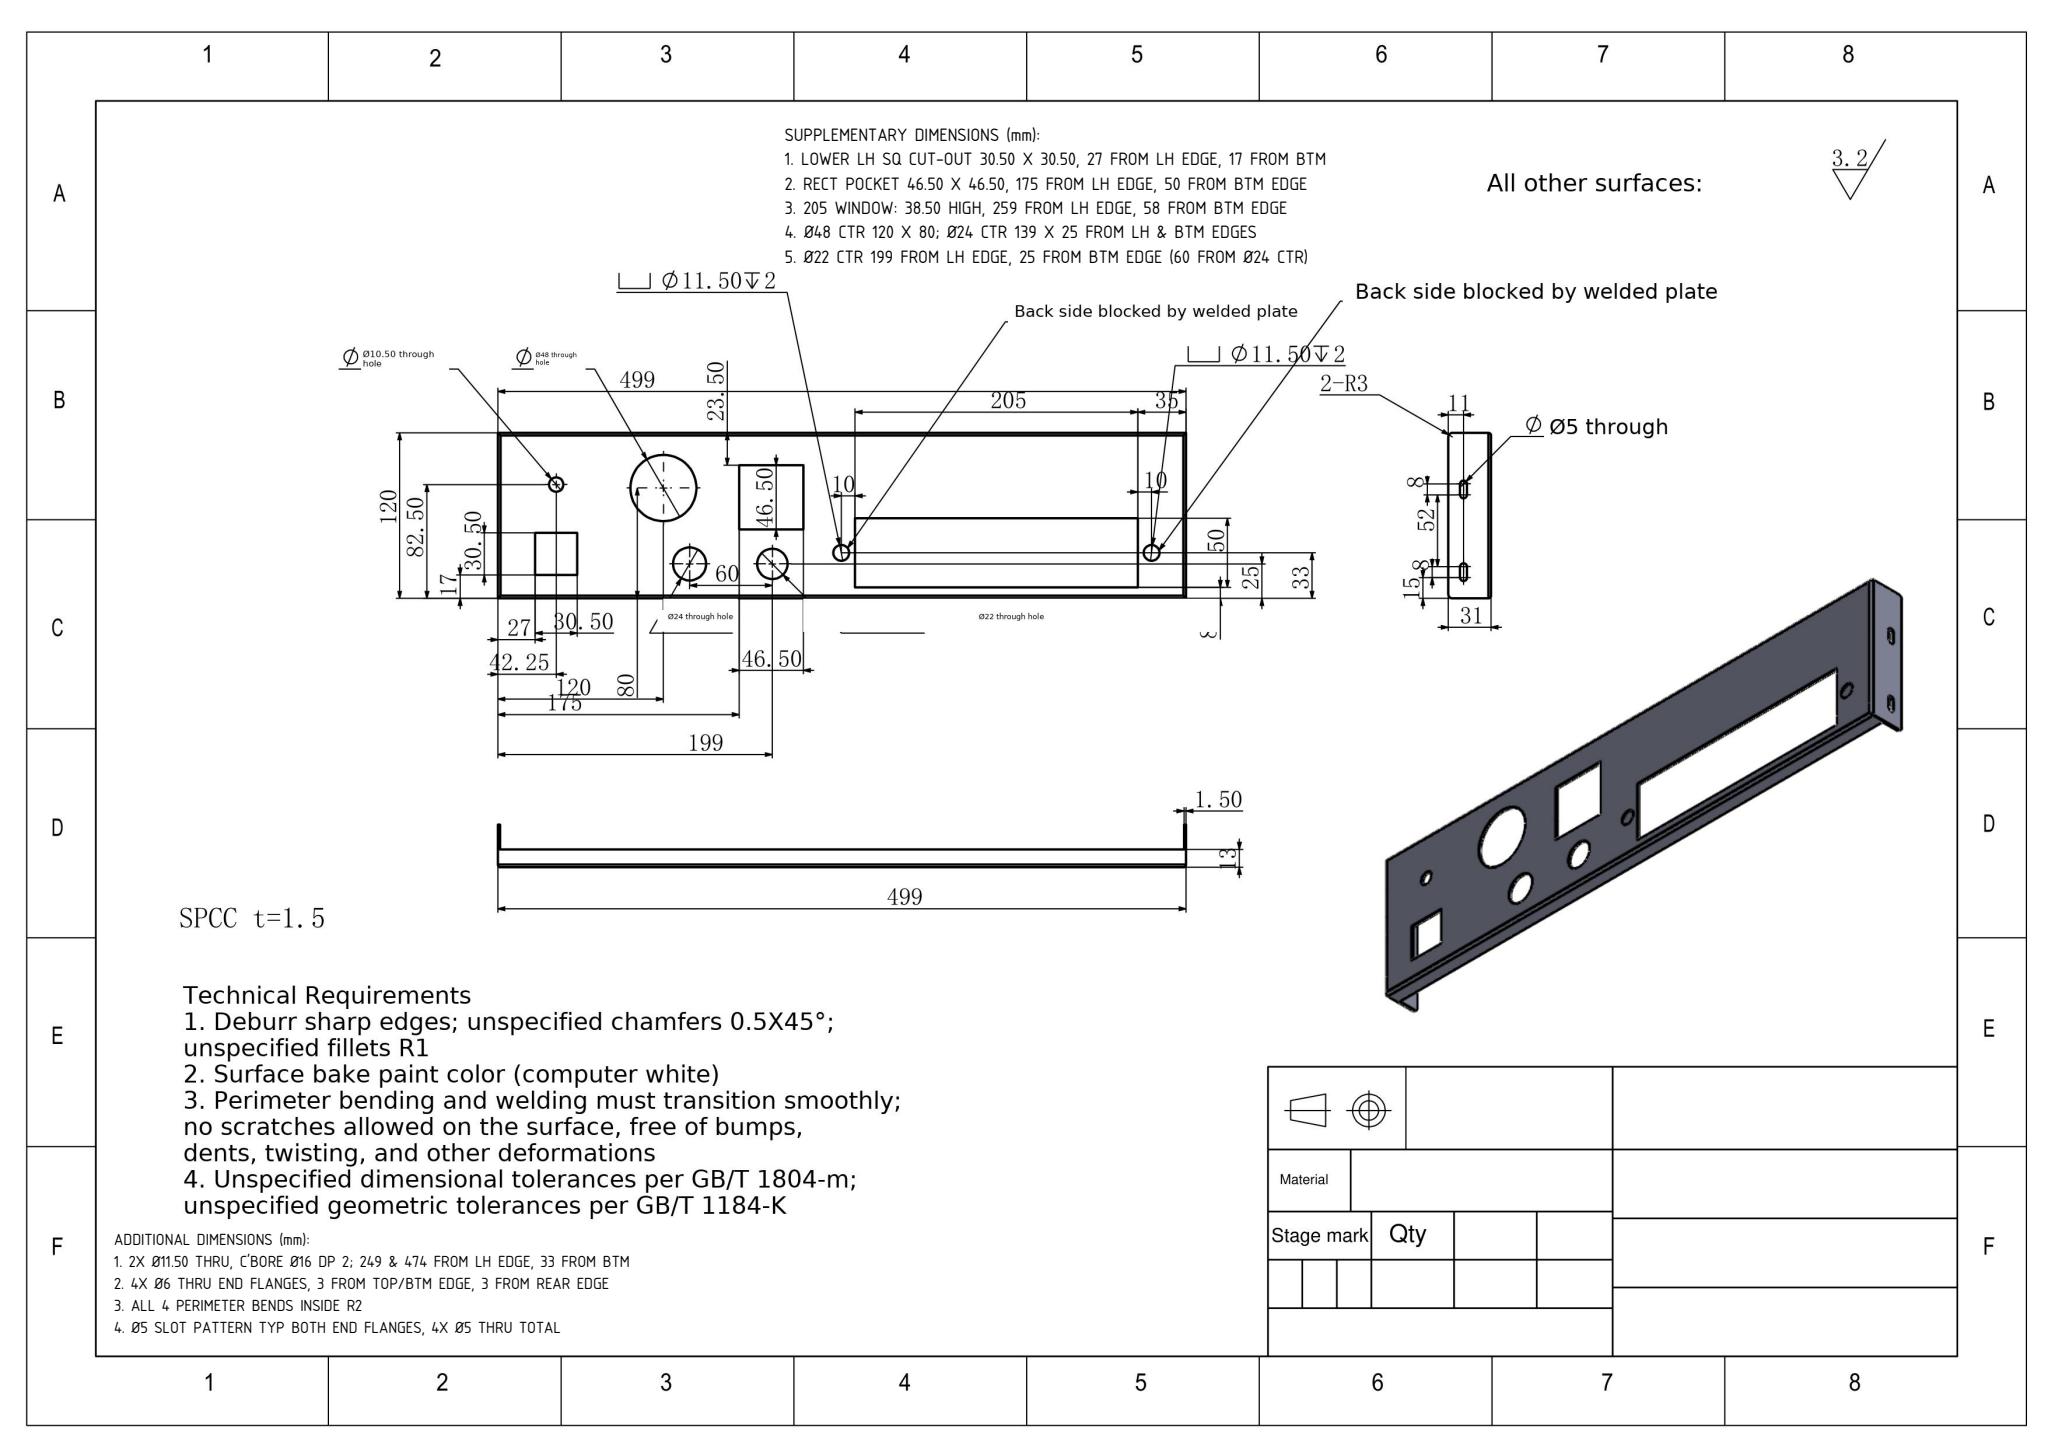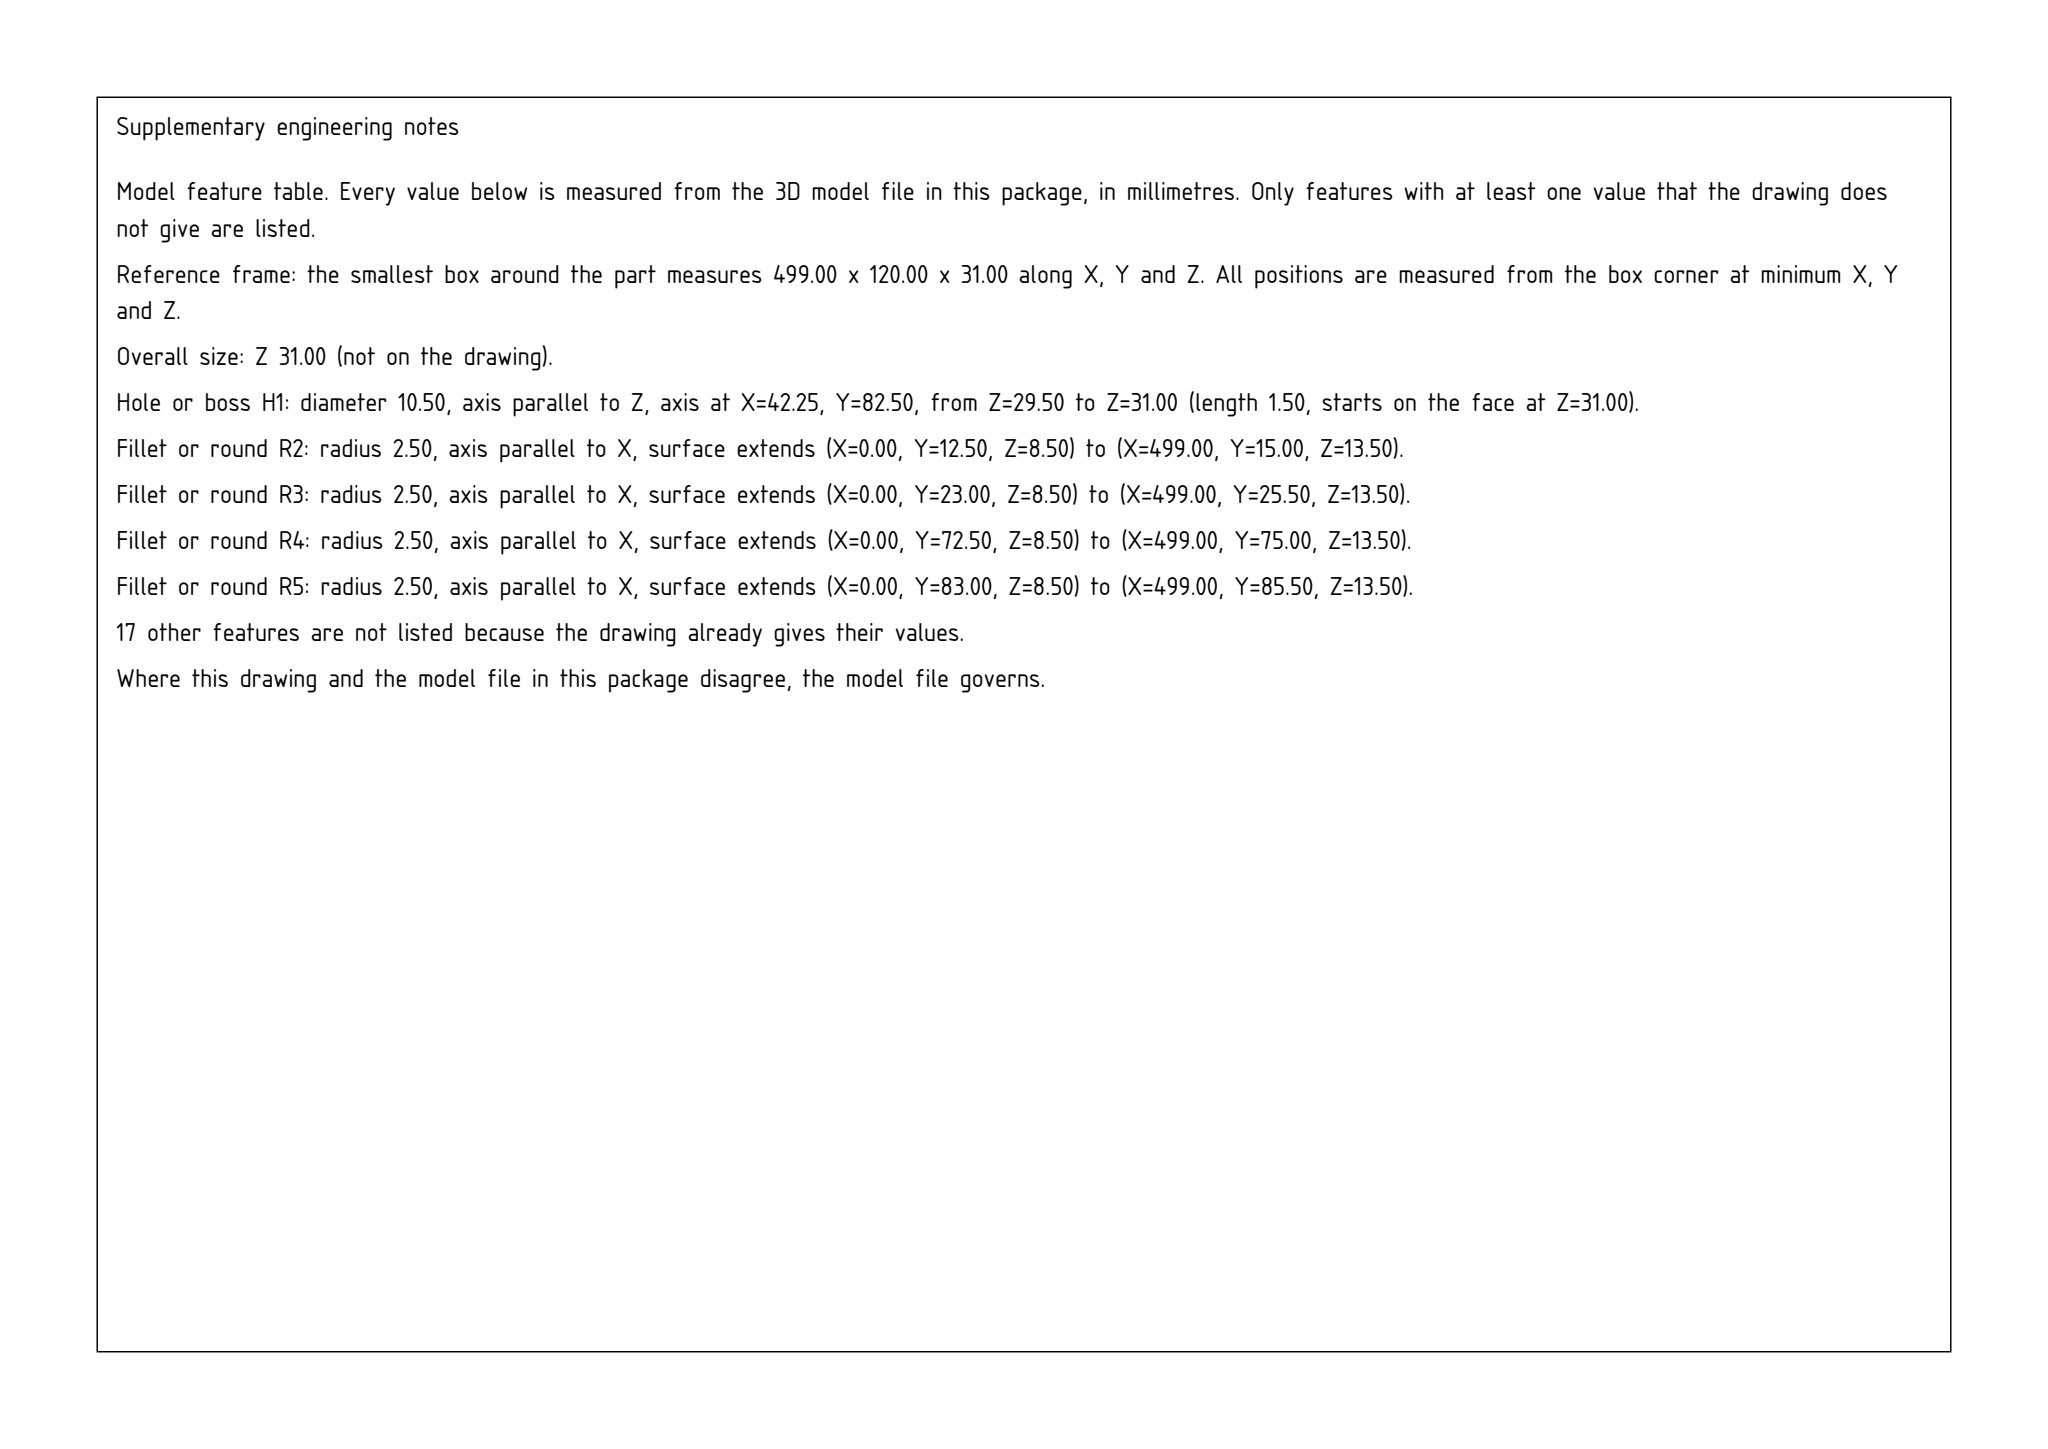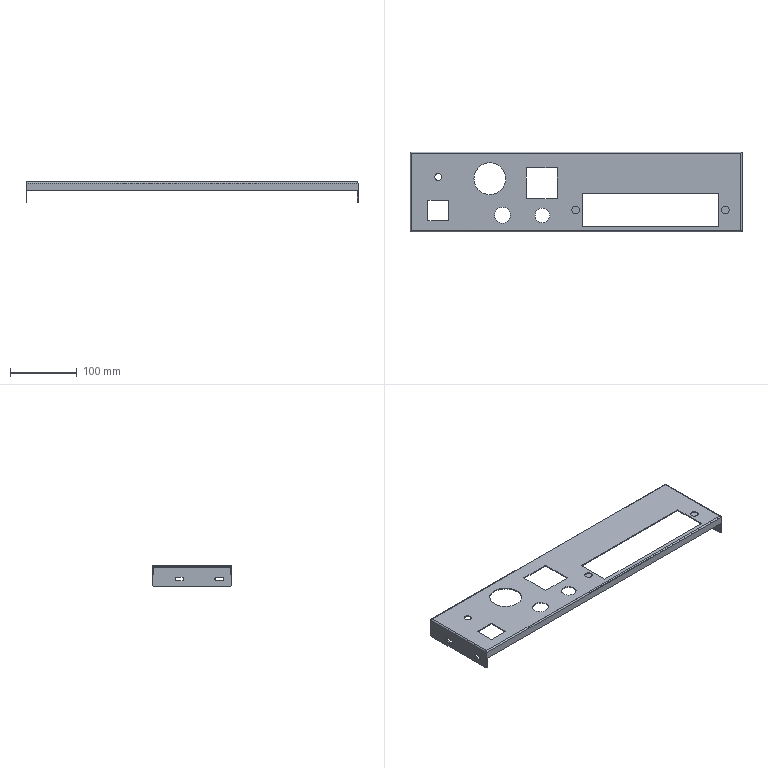Part | SolidWorks | mm | 1 solid | 74 faces | box 499 x 120 x 31 mm | volume 92575 mm3 | plane 38 | cylinder 36 | commonest cylinder face diameters 5 x8 16 x4 11.5 x4 1 x4 4 x4 6 x4 22 x2 24 x2
build123d program:
from build123d import *

# Parameters (mm, degrees)
SKETCH1_W           = 499
SKETCH1_H           = 120
BOSS_EXTRUDE1_DEPTH = 31
SKETCH2_W           = 496
SKETCH2_H           = 15
CUT_EXTRUDE1_DEPTH  = 451.195
SKETCH3_W           = 496
SKETCH3_H           = 96
CUT_EXTRUDE2_DEPTH  = 14.5
SKETCH4_W           = 496
SKETCH4_H           = 13
CUT_EXTRUDE3_DEPTH  = 10.5
SKETCH5_W           = 496
SKETCH5_H           = 13
CUT_EXTRUDE4_DEPTH  = 10.5
CUT_EXTRUDE5_DEPTH  = 620.957
CUT_EXTRUDE6_REACH  = 623.162
CUT_EXTRUDE7_DEPTH  = 620.957
CUT_EXTRUDE8_DEPTH  = 622.162
FILLET1_R           = 0.5
FILLET2_R           = 2
FILLET3_R           = 3
SKETCH10_R          = 5.25
SKETCH10_R_2        = 24
SKETCH10_R_3        = 12
SKETCH10_R_4        = 11
SKETCH10_W          = 30.5
SKETCH10_H          = 30.5
SKETCH10_W_2        = 46.5
SKETCH10_H_2        = 46.5
CUT_EXTRUDE9_DEPTH  = 273.079
SKETCH11_W          = 496
SKETCH11_H          = 120
CUT_EXTRUDE10_DEPTH = 3
SKETCH12_W          = 205
SKETCH12_H          = 50
CUT_EXTRUDE11_DEPTH = 273.079
SKETCH13_R          = 5.75
CUT_EXTRUDE12_DEPTH = 273.079
SKETCH14_R          = 8
BOSS_EXTRUDE2_DEPTH = 2


with BuildPart() as part:
    # Sketch1 → Boss-Extrude1 (new body)
    with BuildSketch(Plane(origin=(0, 0, 324), x_dir=(-1, 0, 0), z_dir=(0, 0, -1))):
        with Locations((0, -44)):
            Rectangle(SKETCH1_W, SKETCH1_H)
    extrude(amount=-BOSS_EXTRUDE1_DEPTH)

    # Sketch2 → Cut-Extrude1 (cut, through all)
    with BuildSketch(Plane(origin=(0, 16, 0), x_dir=(-1, 0, 0), z_dir=(0, 1, 0))):
        with Locations((0, 331.5)):
            Rectangle(SKETCH2_W, SKETCH2_H)
    extrude(amount=-CUT_EXTRUDE1_DEPTH, mode=Mode.SUBTRACT)

    # Sketch3 → Cut-Extrude2 (cut)
    with BuildSketch(Plane(origin=(0, 0, 339), x_dir=(-1, 0, 0), z_dir=(0, 0, -1))):
        with Locations((0, -44)):
            Rectangle(SKETCH3_W, SKETCH3_H)
    extrude(amount=-CUT_EXTRUDE2_DEPTH, mode=Mode.SUBTRACT)

    # Sketch4 → Cut-Extrude3 (cut)
    with BuildSketch(Plane(origin=(0, -92, 0), x_dir=(-1, 0, 0), z_dir=(0, 1, 0))):
        with Locations((0, 347)):
            Rectangle(SKETCH4_W, SKETCH4_H)
    extrude(amount=-CUT_EXTRUDE3_DEPTH, mode=Mode.SUBTRACT)

    # Sketch5 → Cut-Extrude4 (cut)
    with BuildSketch(Plane.XZ.offset(-4)):
        with Locations((0, 347)):
            Rectangle(SKETCH5_W, SKETCH5_H)
    extrude(amount=-CUT_EXTRUDE4_DEPTH, mode=Mode.SUBTRACT)

    # Sketch6 → Cut-Extrude5 (cut, through all)
    with BuildSketch(Plane(origin=(-248, 0, 0), x_dir=(0, 0, -1), z_dir=(1, 0, 0))):
        with BuildLine():
            Line((-332.5, -89), (-332.5, -81))
            ThreePointArc((-332.5, -81), (-335, -78.5), (-337.5, -81))
            Line((-337.5, -81), (-337.5, -89))
            ThreePointArc((-337.5, -89), (-335, -91.5), (-332.5, -89))
        make_face()
    extrude(amount=-CUT_EXTRUDE5_DEPTH, mode=Mode.SUBTRACT)

    # Sketch7 → Cut-Extrude6 (cut, up to next)
    with BuildSketch(Plane.ZY.offset(249.5), mode=Mode.PRIVATE) as cut_extrude6_sk1:
        with BuildLine():
            Line((337.5, -29), (337.5, -21))
            ThreePointArc((337.5, -21), (335, -18.5), (332.5, -21))
            Line((332.5, -21), (332.5, -29))
            ThreePointArc((332.5, -29), (335, -31.5), (337.5, -29))
        make_face()
    cut_extrude6_tool1 = extrude(cut_extrude6_sk1.sketch, amount=-CUT_EXTRUDE6_REACH, mode=Mode.PRIVATE) & part.part
    add(cut_extrude6_tool1.solids().sort_by_distance((-249.5, -25, 335))[0], mode=Mode.SUBTRACT)

    # Sketch8 → Cut-Extrude7 (cut, through all)
    with BuildSketch(Plane.ZY.offset(-248)):
        with BuildLine():
            Line((337.5, -89), (337.5, -81))
            ThreePointArc((337.5, -81), (335, -78.5), (332.5, -81))
            Line((332.5, -81), (332.5, -89))
            ThreePointArc((332.5, -89), (335, -91.5), (337.5, -89))
        make_face()
    extrude(amount=-CUT_EXTRUDE7_DEPTH, mode=Mode.SUBTRACT)

    # Sketch9 → Cut-Extrude8 (cut, through all)
    with BuildSketch(Plane(origin=(249.5, 0, 0), x_dir=(0, 0, -1), z_dir=(1, 0, 0))):
        with BuildLine():
            Line((-332.5, -29), (-332.5, -21))
            ThreePointArc((-332.5, -21), (-335, -18.5), (-337.5, -21))
            Line((-337.5, -21), (-337.5, -29))
            ThreePointArc((-337.5, -29), (-335, -31.5), (-332.5, -29))
        make_face()
    extrude(amount=-CUT_EXTRUDE8_DEPTH, mode=Mode.SUBTRACT)

    # Fillet1
    fillet1_edges = [part.edges().sort_by_distance(p)[0] for p in [
        (248, -44, 353.5),
        (-248, -44, 353.5),
        (0, -102.5, 340.5),
        (0, -102.5, 353.5),
        (0, 14.5, 340.5),
        (0, 14.5, 353.5),
    ]]
    fillet(fillet1_edges, radius=FILLET1_R)

    # Fillet2
    fillet2_edges = [part.edges().sort_by_distance(p)[0] for p in [
        (-249.5, -44, 355),
        (0, 16, 355),
        (0, -104, 339),
        (0, 16, 339),
        (249.5, -44, 355),
        (0, -104, 355),
    ]]
    fillet(fillet2_edges, radius=FILLET2_R)

    # Fillet3
    fillet3_edges = [part.edges().sort_by_distance(p)[0] for p in [
        (-248.75, -104, 324),
        (248.75, 16, 324),
        (-248.75, 16, 324),
        (248.75, -104, 324),
    ]]
    fillet(fillet3_edges, radius=FILLET3_R)

    # Sketch10 → Cut-Extrude9 (cut, through all)
    with BuildSketch(Plane.XY.offset(355)):
        with Locations((-207.25, -21.5)):
            Circle(SKETCH10_R)
        with Locations((-129.5, -24)):
            Circle(SKETCH10_R_2)
        with Locations((-110.5, -79)):
            Circle(SKETCH10_R_3)
        with Locations((-50.5, -79)):
            Circle(SKETCH10_R_4)
        with Locations((-207.25, -71.75)):
            Rectangle(SKETCH10_W, SKETCH10_H)
        with Locations((-51.25, -30.75)):
            Rectangle(SKETCH10_W_2, SKETCH10_H_2)
    extrude(amount=-CUT_EXTRUDE9_DEPTH, mode=Mode.SUBTRACT)

    # Sketch11 → Cut-Extrude10 (cut)
    with BuildSketch(Plane(origin=(0, 0, 339), x_dir=(-1, 0, 0), z_dir=(0, 0, -1))):
        with Locations((0, -44)):
            Rectangle(SKETCH11_W, SKETCH11_H)
    extrude(amount=-CUT_EXTRUDE10_DEPTH, mode=Mode.SUBTRACT)

    # Sketch12 → Cut-Extrude11 (cut, through all)
    with BuildSketch(Plane.XY.offset(355)):
        with Locations((112, -71)):
            Rectangle(SKETCH12_W, SKETCH12_H)
    extrude(amount=-CUT_EXTRUDE11_DEPTH, mode=Mode.SUBTRACT)

    # Sketch13 → Cut-Extrude12 (cut, through all)
    with BuildSketch(Plane.XY.offset(355)):
        with Locations((-0.5, -71)):
            Circle(SKETCH13_R)
        with Locations((224.5, -71)):
            Circle(SKETCH13_R)
    extrude(amount=-CUT_EXTRUDE12_DEPTH, mode=Mode.SUBTRACT)

    # Sketch14 → Boss-Extrude2 (add)
    with BuildSketch(Plane(origin=(0, 0, 353.5), x_dir=(-1, 0, 0), z_dir=(0, 0, -1))):
        with Locations((0.5, -71)):
            Circle(SKETCH14_R)
        with Locations((-224.5, -71)):
            Circle(SKETCH14_R)
    extrude(amount=BOSS_EXTRUDE2_DEPTH)


solid = part.part